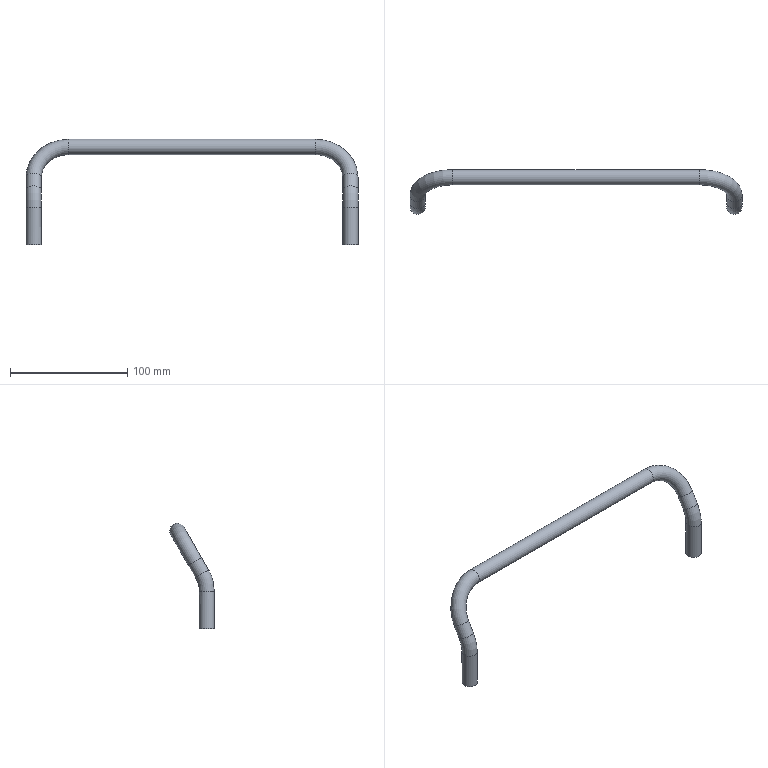Component | NX | METAL_SUPPORT_ROD | 1 solid | 20 faces | volume 22951 mm3 | cylinder 10 | torus 8 | plane 2 | commonest cylinder face diameters 13 x5 10 x5